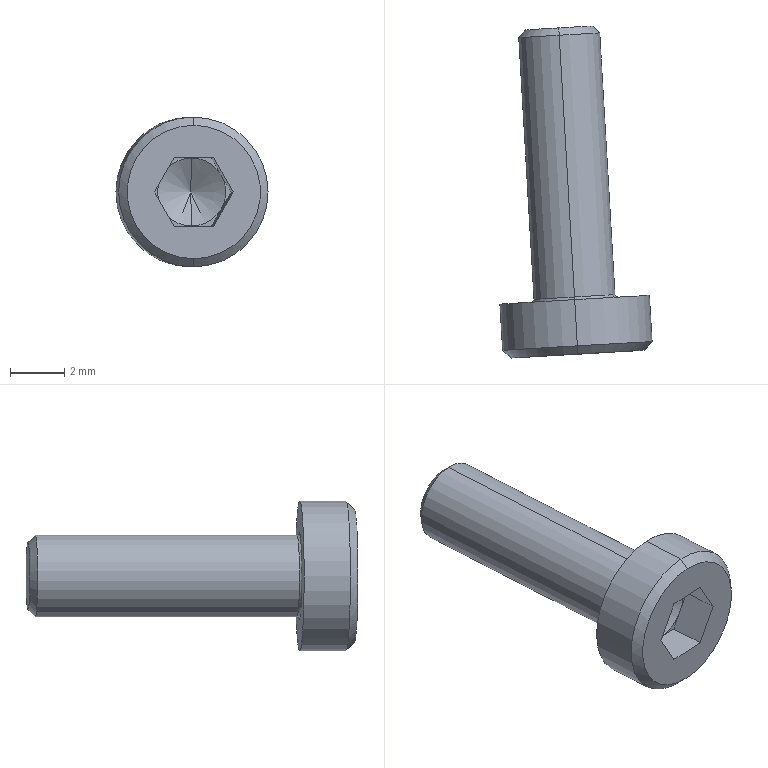Component | SolidWorks | MotorAssemblyWhen2-1_MCOCG20-8-10-1_M3-10_bo2-1 | 1 solid | 27 faces | box 5.59 x 12.19 x 5.5 mm | volume 109 mm3 | plane 15 | cone 6 | cylinder 4 | spline 2 | commonest cylinder face diameters 3 x2 5.5 x2
STEP:
#1=COLOUR_RGB('',0.7922,0.8196,0.9333);
#2=FILL_AREA_STYLE_COLOUR('',#1);
#3=FILL_AREA_STYLE('',(#2));
#4=SURFACE_STYLE_FILL_AREA(#3);
#5=SURFACE_SIDE_STYLE('',(#4));
#6=SURFACE_STYLE_USAGE(.BOTH.,#5);
#7=PRESENTATION_STYLE_ASSIGNMENT((#6));
#8=CARTESIAN_POINT('',(-2.236,5.18,-4.868));
#9=VERTEX_POINT('',#8);
#10=CARTESIAN_POINT('',(-2.236,5.18,-4.986));
#11=VERTEX_POINT('',#10);
#12=CARTESIAN_POINT('',(-2.236,5.18,-4.927));
#13=DIRECTION('',(-0.05821,0.9983,0.));
#14=DIRECTION('',(0.,0.,-1.));
#15=AXIS2_PLACEMENT_3D('',#12,#13,#14);
#16=CIRCLE('',#15,0.05906);
#17=EDGE_CURVE('',#9,#11,#16,.T.);
#18=ORIENTED_EDGE('',*,*,#17,.F.);
#19=CARTESIAN_POINT('',(-2.235,5.176,-4.864));
#20=VERTEX_POINT('',#19);
#21=CARTESIAN_POINT('',(-2.236,5.18,-4.864));
#22=DIRECTION('',(-0.9983,-0.05821,0.));
#23=DIRECTION('',(0.,0.,1.));
#24=AXIS2_PLACEMENT_3D('',#21,#22,#23);
#25=CIRCLE('',#24,0.003937);
#26=EDGE_CURVE('',#9,#20,#25,.T.);
#27=ORIENTED_EDGE('',*,*,#26,.T.);
#28=CARTESIAN_POINT('',(-2.235,5.176,-4.99));
#29=VERTEX_POINT('',#28);
#30=CARTESIAN_POINT('',(-2.235,5.176,-4.99));
#31=CARTESIAN_POINT('',(-2.231,5.176,-4.99));
#32=CARTESIAN_POINT('',(-2.225,5.177,-4.99));
#33=CARTESIAN_POINT('',(-2.219,5.177,-4.988));
#34=CARTESIAN_POINT('',(-2.215,5.177,-4.987));
#35=CARTESIAN_POINT('',(-2.214,5.177,-4.987));
#36=CARTESIAN_POINT('',(-2.213,5.177,-4.986));
#37=CARTESIAN_POINT('',(-2.213,5.177,-4.986));
#38=CARTESIAN_POINT('',(-2.204,5.178,-4.983));
#39=CARTESIAN_POINT('',(-2.197,5.178,-4.978));
#40=CARTESIAN_POINT('',(-2.188,5.179,-4.969));
#41=CARTESIAN_POINT('',(-2.184,5.179,-4.964));
#42=CARTESIAN_POINT('',(-2.18,5.179,-4.957));
#43=CARTESIAN_POINT('',(-2.179,5.179,-4.955));
#44=CARTESIAN_POINT('',(-2.178,5.179,-4.953));
#45=CARTESIAN_POINT('',(-2.177,5.179,-4.951));
#46=CARTESIAN_POINT('',(-2.174,5.18,-4.943));
#47=CARTESIAN_POINT('',(-2.172,5.18,-4.935));
#48=CARTESIAN_POINT('',(-2.172,5.18,-4.923));
#49=CARTESIAN_POINT('',(-2.173,5.18,-4.917));
#50=CARTESIAN_POINT('',(-2.175,5.179,-4.911));
#51=CARTESIAN_POINT('',(-2.176,5.179,-4.907));
#52=CARTESIAN_POINT('',(-2.176,5.179,-4.906));
#53=CARTESIAN_POINT('',(-2.176,5.179,-4.905));
#54=CARTESIAN_POINT('',(-2.177,5.179,-4.905));
#55=CARTESIAN_POINT('',(-2.18,5.179,-4.896));
#56=CARTESIAN_POINT('',(-2.185,5.179,-4.889));
#57=CARTESIAN_POINT('',(-2.194,5.178,-4.88));
#58=CARTESIAN_POINT('',(-2.199,5.178,-4.876));
#59=CARTESIAN_POINT('',(-2.205,5.178,-4.872));
#60=CARTESIAN_POINT('',(-2.208,5.178,-4.871));
#61=CARTESIAN_POINT('',(-2.21,5.177,-4.87));
#62=CARTESIAN_POINT('',(-2.211,5.177,-4.869));
#63=CARTESIAN_POINT('',(-2.22,5.177,-4.866));
#64=CARTESIAN_POINT('',(-2.227,5.176,-4.864));
#65=CARTESIAN_POINT('',(-2.235,5.176,-4.864));
#66=B_SPLINE_CURVE_WITH_KNOTS('',3,(#30,#31,#32,#33,#34,#35,#36,#37,#38,#39,#40,#41,#42,#43,#44,#45,#46,#47,#48,#49,#50,#51,#52,#53,#54,#55,#56,#57,#58,#59,#60,#61,#62,#63,#64,#65),.UNSPECIFIED.,.F.,.F.,(4,1,1,1,2,2,2,1,1,2,2,2,1,1,1,2,2,2,1,1,2,2,4),(0.,0.0625,0.09375,0.1094,0.1172,0.125,0.25,0.3125,0.3438,0.3594,0.375,0.5,0.5625,0.5938,0.6094,0.6172,0.625,0.75,0.8125,0.8438,0.8594,0.875,1.),.UNSPECIFIED.);
#67=EDGE_CURVE('',#29,#20,#66,.T.);
#68=ORIENTED_EDGE('',*,*,#67,.F.);
#69=CARTESIAN_POINT('',(-2.236,5.18,-4.99));
#70=DIRECTION('',(0.9983,0.05821,0.));
#71=DIRECTION('',(0.,0.,-1.));
#72=AXIS2_PLACEMENT_3D('',#69,#70,#71);
#73=CIRCLE('',#72,0.003937);
#74=EDGE_CURVE('',#11,#29,#73,.T.);
#75=ORIENTED_EDGE('',*,*,#74,.F.);
#76=EDGE_LOOP('',(#18,#27,#68,#75));
#77=FACE_OUTER_BOUND('',#76,.T.);
#78=CARTESIAN_POINT('',(-2.236,5.18,-4.986));
#79=CARTESIAN_POINT('',(-2.118,5.187,-4.986));
#80=CARTESIAN_POINT('',(-2.118,5.187,-4.868));
#81=CARTESIAN_POINT('',(-2.236,5.18,-4.868));
#82=CARTESIAN_POINT('',(-2.235,5.178,-4.986));
#83=CARTESIAN_POINT('',(-2.117,5.184,-4.986));
#84=CARTESIAN_POINT('',(-2.117,5.184,-4.868));
#85=CARTESIAN_POINT('',(-2.235,5.178,-4.868));
#86=CARTESIAN_POINT('',(-2.235,5.176,-4.988));
#87=CARTESIAN_POINT('',(-2.114,5.183,-4.988));
#88=CARTESIAN_POINT('',(-2.114,5.183,-4.867));
#89=CARTESIAN_POINT('',(-2.235,5.176,-4.867));
#90=CARTESIAN_POINT('',(-2.235,5.176,-4.99));
#91=CARTESIAN_POINT('',(-2.11,5.183,-4.99));
#92=CARTESIAN_POINT('',(-2.11,5.183,-4.864));
#93=CARTESIAN_POINT('',(-2.235,5.176,-4.864));
#94=(BOUNDED_SURFACE()B_SPLINE_SURFACE(3,3,((#78,#79,#80,#81),(#82,#83,#84,#85),(#86,#87,#88,#89),(#90,#91,#92,#93)),.UNSPECIFIED.,.F.,.F.,.T.)B_SPLINE_SURFACE_WITH_KNOTS((4,4),(4,4),(0.,1.),(0.,1.),.UNSPECIFIED.)GEOMETRIC_REPRESENTATION_ITEM()RATIONAL_B_SPLINE_SURFACE(((1.,0.3333,0.3333,1.),(0.8047,0.2682,0.2682,0.8047),(0.8047,0.2682,0.2682,0.8047),(1.,0.3333,0.3333,1.)))REPRESENTATION_ITEM('')SURFACE());
#95=ADVANCED_FACE('',(#77),#94,.F.);
#96=CARTESIAN_POINT('',(-2.258,5.558,-4.986));
#97=VERTEX_POINT('',#96);
#98=CARTESIAN_POINT('',(-2.258,5.558,-4.868));
#99=VERTEX_POINT('',#98);
#100=CARTESIAN_POINT('',(-2.258,5.558,-4.927));
#101=DIRECTION('',(0.05821,-0.9983,-0.));
#102=DIRECTION('',(0.,0.,-1.));
#103=AXIS2_PLACEMENT_3D('',#100,#101,#102);
#104=CIRCLE('',#103,0.05906);
#105=EDGE_CURVE('',#97,#99,#104,.T.);
#106=ORIENTED_EDGE('',*,*,#105,.T.);
#107=CARTESIAN_POINT('',(-2.258,5.569,-4.868));
#108=DIRECTION('',(0.05821,-0.9983,-0.));
#109=VECTOR('',#108,39.37);
#110=LINE('',#107,#109);
#111=EDGE_CURVE('',#99,#9,#110,.T.);
#112=ORIENTED_EDGE('',*,*,#111,.T.);
#113=ORIENTED_EDGE('',*,*,#17,.T.);
#114=CARTESIAN_POINT('',(-2.258,5.569,-4.986));
#115=DIRECTION('',(0.05821,-0.9983,-0.));
#116=VECTOR('',#115,39.37);
#117=LINE('',#114,#116);
#118=EDGE_CURVE('',#97,#11,#117,.T.);
#119=ORIENTED_EDGE('',*,*,#118,.F.);
#120=EDGE_LOOP('',(#106,#112,#113,#119));
#121=FACE_OUTER_BOUND('',#120,.T.);
#122=CARTESIAN_POINT('',(-2.258,5.569,-4.927));
#123=DIRECTION('',(0.05821,-0.9983,-0.));
#124=DIRECTION('',(0.,0.,-1.));
#125=AXIS2_PLACEMENT_3D('',#122,#123,#124);
#126=CYLINDRICAL_SURFACE('',#125,0.05906);
#127=ADVANCED_FACE('',(#121),#126,.T.);
#128=CARTESIAN_POINT('',(-2.258,5.569,-4.976));
#129=VERTEX_POINT('',#128);
#130=CARTESIAN_POINT('',(-2.258,5.569,-4.879));
#131=VERTEX_POINT('',#130);
#132=CARTESIAN_POINT('',(-2.258,5.569,-4.927));
#133=DIRECTION('',(0.05821,-0.9983,-0.));
#134=DIRECTION('',(0.,0.,-1.));
#135=AXIS2_PLACEMENT_3D('',#132,#133,#134);
#136=CIRCLE('',#135,0.04841);
#137=EDGE_CURVE('',#129,#131,#136,.T.);
#138=ORIENTED_EDGE('',*,*,#137,.T.);
#139=CARTESIAN_POINT('',(-2.258,5.558,-4.868));
#140=DIRECTION('',(0.04116,-0.7059,0.7071));
#141=VECTOR('',#140,39.37);
#142=LINE('',#139,#141);
#143=EDGE_CURVE('',#131,#99,#142,.T.);
#144=ORIENTED_EDGE('',*,*,#143,.T.);
#145=ORIENTED_EDGE('',*,*,#105,.F.);
#146=CARTESIAN_POINT('',(-2.258,5.558,-4.986));
#147=DIRECTION('',(0.04116,-0.7059,-0.7071));
#148=VECTOR('',#147,39.37);
#149=LINE('',#146,#148);
#150=EDGE_CURVE('',#129,#97,#149,.T.);
#151=ORIENTED_EDGE('',*,*,#150,.F.);
#152=EDGE_LOOP('',(#138,#144,#145,#151));
#153=FACE_OUTER_BOUND('',#152,.T.);
#154=CARTESIAN_POINT('',(-2.258,5.558,-4.927));
#155=DIRECTION('',(0.05821,-0.9983,-0.));
#156=DIRECTION('',(0.,0.,-1.));
#157=AXIS2_PLACEMENT_3D('',#154,#155,#156);
#158=CONICAL_SURFACE('',#157,0.05906,0.7854);
#159=ADVANCED_FACE('',(#153),#158,.T.);
#160=CARTESIAN_POINT('',(-2.235,5.176,-5.036));
#161=VERTEX_POINT('',#160);
#162=CARTESIAN_POINT('',(-2.235,5.176,-4.819));
#163=VERTEX_POINT('',#162);
#164=CARTESIAN_POINT('',(-2.235,5.176,-4.927));
#165=DIRECTION('',(0.05821,-0.9983,-0.));
#166=DIRECTION('',(0.,0.,-1.));
#167=AXIS2_PLACEMENT_3D('',#164,#165,#166);
#168=CIRCLE('',#167,0.1083);
#169=EDGE_CURVE('',#161,#163,#168,.T.);
#170=ORIENTED_EDGE('',*,*,#169,.T.);
#171=CARTESIAN_POINT('',(-2.231,5.109,-4.819));
#172=VERTEX_POINT('',#171);
#173=CARTESIAN_POINT('',(-2.258,5.569,-4.819));
#174=DIRECTION('',(0.05821,-0.9983,-0.));
#175=VECTOR('',#174,39.37);
#176=LINE('',#173,#175);
#177=EDGE_CURVE('',#163,#172,#176,.T.);
#178=ORIENTED_EDGE('',*,*,#177,.T.);
#179=CARTESIAN_POINT('',(-2.231,5.109,-5.036));
#180=VERTEX_POINT('',#179);
#181=CARTESIAN_POINT('',(-2.231,5.109,-4.927));
#182=DIRECTION('',(-0.05821,0.9983,0.));
#183=DIRECTION('',(-0.,0.,-1.));
#184=AXIS2_PLACEMENT_3D('',#181,#182,#183);
#185=CIRCLE('',#184,0.1083);
#186=EDGE_CURVE('',#172,#180,#185,.T.);
#187=ORIENTED_EDGE('',*,*,#186,.T.);
#188=CARTESIAN_POINT('',(-2.258,5.569,-5.036));
#189=DIRECTION('',(0.05821,-0.9983,-0.));
#190=VECTOR('',#189,39.37);
#191=LINE('',#188,#190);
#192=EDGE_CURVE('',#161,#180,#191,.T.);
#193=ORIENTED_EDGE('',*,*,#192,.F.);
#194=EDGE_LOOP('',(#170,#178,#187,#193));
#195=FACE_OUTER_BOUND('',#194,.T.);
#196=CARTESIAN_POINT('',(-2.258,5.569,-4.927));
#197=DIRECTION('',(0.05821,-0.9983,-0.));
#198=DIRECTION('',(0.,0.,-1.));
#199=AXIS2_PLACEMENT_3D('',#196,#197,#198);
#200=CYLINDRICAL_SURFACE('',#199,0.1083);
#201=ADVANCED_FACE('',(#195),#200,.T.);
#202=CARTESIAN_POINT('',(-2.231,5.097,-4.831));
#203=VERTEX_POINT('',#202);
#204=CARTESIAN_POINT('',(-2.231,5.097,-5.024));
#205=VERTEX_POINT('',#204);
#206=CARTESIAN_POINT('',(-2.231,5.097,-4.927));
#207=DIRECTION('',(-0.05821,0.9983,0.));
#208=DIRECTION('',(0.,0.,1.));
#209=AXIS2_PLACEMENT_3D('',#206,#207,#208);
#210=CIRCLE('',#209,0.09646);
#211=EDGE_CURVE('',#203,#205,#210,.T.);
#212=ORIENTED_EDGE('',*,*,#211,.T.);
#213=CARTESIAN_POINT('',(-2.231,5.109,-5.036));
#214=DIRECTION('',(-0.04116,0.7059,-0.7071));
#215=VECTOR('',#214,39.37);
#216=LINE('',#213,#215);
#217=EDGE_CURVE('',#205,#180,#216,.T.);
#218=ORIENTED_EDGE('',*,*,#217,.T.);
#219=ORIENTED_EDGE('',*,*,#186,.F.);
#220=CARTESIAN_POINT('',(-2.231,5.109,-4.819));
#221=DIRECTION('',(-0.04116,0.7059,0.7071));
#222=VECTOR('',#221,39.37);
#223=LINE('',#220,#222);
#224=EDGE_CURVE('',#203,#172,#223,.T.);
#225=ORIENTED_EDGE('',*,*,#224,.F.);
#226=EDGE_LOOP('',(#212,#218,#219,#225));
#227=FACE_OUTER_BOUND('',#226,.T.);
#228=CARTESIAN_POINT('',(-2.231,5.109,-4.927));
#229=DIRECTION('',(-0.05821,0.9983,0.));
#230=DIRECTION('',(0.,0.,1.));
#231=AXIS2_PLACEMENT_3D('',#228,#229,#230);
#232=CONICAL_SURFACE('',#231,0.1083,0.7854);
#233=ADVANCED_FACE('',(#227),#232,.T.);
#234=CARTESIAN_POINT('',(-2.235,5.177,-4.927));
#235=VERTEX_POINT('',#234);
#236=CARTESIAN_POINT('',(-2.234,5.148,-4.977));
#237=VERTEX_POINT('',#236);
#238=CARTESIAN_POINT('',(-2.234,5.148,-4.977));
#239=DIRECTION('',(0.0291,-0.4992,-0.866));
#240=VECTOR('',#239,39.37);
#241=LINE('',#238,#240);
#242=EDGE_CURVE('',#235,#237,#241,.T.);
#243=ORIENTED_EDGE('',*,*,#242,.F.);
#244=CARTESIAN_POINT('',(-2.234,5.148,-4.878));
#245=VERTEX_POINT('',#244);
#246=CARTESIAN_POINT('',(-2.234,5.148,-4.878));
#247=DIRECTION('',(0.0291,-0.4992,0.866));
#248=VECTOR('',#247,39.37);
#249=LINE('',#246,#248);
#250=EDGE_CURVE('',#235,#245,#249,.T.);
#251=ORIENTED_EDGE('',*,*,#250,.T.);
#252=CARTESIAN_POINT('',(-2.276,5.146,-4.903));
#253=VERTEX_POINT('',#252);
#254=CARTESIAN_POINT('',(-2.234,5.148,-4.927));
#255=DIRECTION('',(0.05821,-0.9983,-0.));
#256=DIRECTION('',(0.,0.,-1.));
#257=AXIS2_PLACEMENT_3D('',#254,#255,#256);
#258=CIRCLE('',#257,0.04921);
#259=EDGE_CURVE('',#245,#253,#258,.T.);
#260=ORIENTED_EDGE('',*,*,#259,.T.);
#261=CARTESIAN_POINT('',(-2.276,5.146,-4.952));
#262=VERTEX_POINT('',#261);
#263=CARTESIAN_POINT('',(-2.234,5.148,-4.927));
#264=DIRECTION('',(0.05821,-0.9983,-0.));
#265=DIRECTION('',(0.,0.,-1.));
#266=AXIS2_PLACEMENT_3D('',#263,#264,#265);
#267=CIRCLE('',#266,0.04921);
#268=EDGE_CURVE('',#253,#262,#267,.T.);
#269=ORIENTED_EDGE('',*,*,#268,.T.);
#270=CARTESIAN_POINT('',(-2.234,5.148,-4.927));
#271=DIRECTION('',(0.05821,-0.9983,-0.));
#272=DIRECTION('',(0.,0.,-1.));
#273=AXIS2_PLACEMENT_3D('',#270,#271,#272);
#274=CIRCLE('',#273,0.04921);
#275=EDGE_CURVE('',#262,#237,#274,.T.);
#276=ORIENTED_EDGE('',*,*,#275,.T.);
#277=EDGE_LOOP('',(#243,#251,#260,#269,#276));
#278=FACE_OUTER_BOUND('',#277,.T.);
#279=CARTESIAN_POINT('',(-2.234,5.148,-4.927));
#280=DIRECTION('',(0.05821,-0.9983,-0.));
#281=DIRECTION('',(0.,0.,-1.));
#282=AXIS2_PLACEMENT_3D('',#279,#280,#281);
#283=CONICAL_SURFACE('',#282,0.04921,1.047);
#284=ADVANCED_FACE('',(#278),#283,.F.);
#285=ORIENTED_EDGE('',*,*,#111,.F.);
#286=CARTESIAN_POINT('',(-2.258,5.558,-4.927));
#287=DIRECTION('',(0.05821,-0.9983,-0.));
#288=DIRECTION('',(0.,0.,-1.));
#289=AXIS2_PLACEMENT_3D('',#286,#287,#288);
#290=CIRCLE('',#289,0.05906);
#291=EDGE_CURVE('',#99,#97,#290,.T.);
#292=ORIENTED_EDGE('',*,*,#291,.T.);
#293=ORIENTED_EDGE('',*,*,#118,.T.);
#294=CARTESIAN_POINT('',(-2.236,5.18,-4.927));
#295=DIRECTION('',(-0.05821,0.9983,0.));
#296=DIRECTION('',(0.,0.,-1.));
#297=AXIS2_PLACEMENT_3D('',#294,#295,#296);
#298=CIRCLE('',#297,0.05906);
#299=EDGE_CURVE('',#11,#9,#298,.T.);
#300=ORIENTED_EDGE('',*,*,#299,.T.);
#301=EDGE_LOOP('',(#285,#292,#293,#300));
#302=FACE_OUTER_BOUND('',#301,.T.);
#303=CARTESIAN_POINT('',(-2.258,5.569,-4.927));
#304=DIRECTION('',(0.05821,-0.9983,-0.));
#305=DIRECTION('',(0.,0.,-1.));
#306=AXIS2_PLACEMENT_3D('',#303,#304,#305);
#307=CYLINDRICAL_SURFACE('',#306,0.05906);
#308=ADVANCED_FACE('',(#302),#307,.T.);
#309=ORIENTED_EDGE('',*,*,#26,.F.);
#310=ORIENTED_EDGE('',*,*,#299,.F.);
#311=ORIENTED_EDGE('',*,*,#74,.T.);
#312=CARTESIAN_POINT('',(-2.235,5.176,-4.864));
#313=CARTESIAN_POINT('',(-2.239,5.176,-4.864));
#314=CARTESIAN_POINT('',(-2.245,5.175,-4.865));
#315=CARTESIAN_POINT('',(-2.252,5.175,-4.867));
#316=CARTESIAN_POINT('',(-2.255,5.175,-4.868));
#317=CARTESIAN_POINT('',(-2.257,5.175,-4.868));
#318=CARTESIAN_POINT('',(-2.258,5.175,-4.868));
#319=CARTESIAN_POINT('',(-2.258,5.175,-4.869));
#320=CARTESIAN_POINT('',(-2.267,5.174,-4.872));
#321=CARTESIAN_POINT('',(-2.274,5.174,-4.877));
#322=CARTESIAN_POINT('',(-2.283,5.173,-4.886));
#323=CARTESIAN_POINT('',(-2.287,5.173,-4.891));
#324=CARTESIAN_POINT('',(-2.291,5.173,-4.897));
#325=CARTESIAN_POINT('',(-2.292,5.173,-4.9));
#326=CARTESIAN_POINT('',(-2.293,5.173,-4.902));
#327=CARTESIAN_POINT('',(-2.293,5.173,-4.903));
#328=CARTESIAN_POINT('',(-2.297,5.172,-4.912));
#329=CARTESIAN_POINT('',(-2.298,5.172,-4.919));
#330=CARTESIAN_POINT('',(-2.298,5.172,-4.931));
#331=CARTESIAN_POINT('',(-2.298,5.172,-4.937));
#332=CARTESIAN_POINT('',(-2.296,5.172,-4.944));
#333=CARTESIAN_POINT('',(-2.295,5.172,-4.947));
#334=CARTESIAN_POINT('',(-2.294,5.172,-4.949));
#335=CARTESIAN_POINT('',(-2.294,5.173,-4.95));
#336=CARTESIAN_POINT('',(-2.294,5.173,-4.95));
#337=CARTESIAN_POINT('',(-2.291,5.173,-4.959));
#338=CARTESIAN_POINT('',(-2.286,5.173,-4.966));
#339=CARTESIAN_POINT('',(-2.277,5.174,-4.975));
#340=CARTESIAN_POINT('',(-2.272,5.174,-4.979));
#341=CARTESIAN_POINT('',(-2.265,5.174,-4.983));
#342=CARTESIAN_POINT('',(-2.262,5.174,-4.984));
#343=CARTESIAN_POINT('',(-2.26,5.174,-4.985));
#344=CARTESIAN_POINT('',(-2.259,5.175,-4.986));
#345=CARTESIAN_POINT('',(-2.251,5.175,-4.989));
#346=CARTESIAN_POINT('',(-2.243,5.175,-4.99));
#347=CARTESIAN_POINT('',(-2.235,5.176,-4.99));
#348=B_SPLINE_CURVE_WITH_KNOTS('',3,(#312,#313,#314,#315,#316,#317,#318,#319,#320,#321,#322,#323,#324,#325,#326,#327,#328,#329,#330,#331,#332,#333,#334,#335,#336,#337,#338,#339,#340,#341,#342,#343,#344,#345,#346,#347),.UNSPECIFIED.,.F.,.F.,(4,1,1,1,2,2,2,1,1,2,2,2,1,1,1,2,2,2,1,1,2,2,4),(0.,0.0625,0.09375,0.1094,0.1172,0.125,0.25,0.3125,0.3438,0.3594,0.375,0.5,0.5625,0.5938,0.6094,0.6172,0.625,0.75,0.8125,0.8438,0.8594,0.875,1.),.UNSPECIFIED.);
#349=EDGE_CURVE('',#20,#29,#348,.T.);
#350=ORIENTED_EDGE('',*,*,#349,.F.);
#351=EDGE_LOOP('',(#309,#310,#311,#350));
#352=FACE_OUTER_BOUND('',#351,.T.);
#353=CARTESIAN_POINT('',(-2.236,5.18,-4.868));
#354=CARTESIAN_POINT('',(-2.353,5.173,-4.868));
#355=CARTESIAN_POINT('',(-2.353,5.173,-4.986));
#356=CARTESIAN_POINT('',(-2.236,5.18,-4.986));
#357=CARTESIAN_POINT('',(-2.235,5.178,-4.868));
#358=CARTESIAN_POINT('',(-2.353,5.171,-4.868));
#359=CARTESIAN_POINT('',(-2.353,5.171,-4.986));
#360=CARTESIAN_POINT('',(-2.235,5.178,-4.986));
#361=CARTESIAN_POINT('',(-2.235,5.176,-4.867));
#362=CARTESIAN_POINT('',(-2.356,5.169,-4.867));
#363=CARTESIAN_POINT('',(-2.356,5.169,-4.988));
#364=CARTESIAN_POINT('',(-2.235,5.176,-4.988));
#365=CARTESIAN_POINT('',(-2.235,5.176,-4.864));
#366=CARTESIAN_POINT('',(-2.361,5.169,-4.864));
#367=CARTESIAN_POINT('',(-2.361,5.169,-4.99));
#368=CARTESIAN_POINT('',(-2.235,5.176,-4.99));
#369=(BOUNDED_SURFACE()B_SPLINE_SURFACE(3,3,((#353,#354,#355,#356),(#357,#358,#359,#360),(#361,#362,#363,#364),(#365,#366,#367,#368)),.UNSPECIFIED.,.F.,.F.,.T.)B_SPLINE_SURFACE_WITH_KNOTS((4,4),(4,4),(0.,1.),(0.,1.),.UNSPECIFIED.)GEOMETRIC_REPRESENTATION_ITEM()RATIONAL_B_SPLINE_SURFACE(((1.,0.3333,0.3333,1.),(0.8047,0.2682,0.2682,0.8047),(0.8047,0.2682,0.2682,0.8047),(1.,0.3333,0.3333,1.)))REPRESENTATION_ITEM('')SURFACE());
#370=ADVANCED_FACE('',(#352),#369,.F.);
#371=ORIENTED_EDGE('',*,*,#143,.F.);
#372=CARTESIAN_POINT('',(-2.258,5.569,-4.927));
#373=DIRECTION('',(0.05821,-0.9983,-0.));
#374=DIRECTION('',(0.,0.,-1.));
#375=AXIS2_PLACEMENT_3D('',#372,#373,#374);
#376=CIRCLE('',#375,0.04841);
#377=EDGE_CURVE('',#131,#129,#376,.T.);
#378=ORIENTED_EDGE('',*,*,#377,.T.);
#379=ORIENTED_EDGE('',*,*,#150,.T.);
#380=ORIENTED_EDGE('',*,*,#291,.F.);
#381=EDGE_LOOP('',(#371,#378,#379,#380));
#382=FACE_OUTER_BOUND('',#381,.T.);
#383=CARTESIAN_POINT('',(-2.258,5.558,-4.927));
#384=DIRECTION('',(0.05821,-0.9983,-0.));
#385=DIRECTION('',(0.,0.,-1.));
#386=AXIS2_PLACEMENT_3D('',#383,#384,#385);
#387=CONICAL_SURFACE('',#386,0.05906,0.7854);
#388=ADVANCED_FACE('',(#382),#387,.T.);
#389=ORIENTED_EDGE('',*,*,#349,.T.);
#390=ORIENTED_EDGE('',*,*,#67,.T.);
#391=EDGE_LOOP('',(#389,#390));
#392=FACE_BOUND('',#391,.T.);
#393=ORIENTED_EDGE('',*,*,#169,.F.);
#394=CARTESIAN_POINT('',(-2.235,5.176,-4.927));
#395=DIRECTION('',(0.05821,-0.9983,-0.));
#396=DIRECTION('',(0.,0.,-1.));
#397=AXIS2_PLACEMENT_3D('',#394,#395,#396);
#398=CIRCLE('',#397,0.1083);
#399=EDGE_CURVE('',#163,#161,#398,.T.);
#400=ORIENTED_EDGE('',*,*,#399,.F.);
#401=EDGE_LOOP('',(#393,#400));
#402=FACE_OUTER_BOUND('',#401,.T.);
#403=CARTESIAN_POINT('',(-2.127,5.182,-4.927));
#404=DIRECTION('',(0.05821,-0.9983,-0.));
#405=DIRECTION('',(-0.,0.,-1.));
#406=AXIS2_PLACEMENT_3D('',#403,#404,#405);
#407=PLANE('',#406);
#408=ADVANCED_FACE('',(#392,#402),#407,.F.);
#409=ORIENTED_EDGE('',*,*,#137,.F.);
#410=ORIENTED_EDGE('',*,*,#377,.F.);
#411=EDGE_LOOP('',(#409,#410));
#412=FACE_OUTER_BOUND('',#411,.T.);
#413=CARTESIAN_POINT('',(-2.21,5.572,-4.927));
#414=DIRECTION('',(0.05821,-0.9983,-0.));
#415=DIRECTION('',(-0.,0.,-1.));
#416=AXIS2_PLACEMENT_3D('',#413,#414,#415);
#417=PLANE('',#416);
#418=ADVANCED_FACE('',(#412),#417,.F.);
#419=ORIENTED_EDGE('',*,*,#177,.F.);
#420=ORIENTED_EDGE('',*,*,#399,.T.);
#421=ORIENTED_EDGE('',*,*,#192,.T.);
#422=CARTESIAN_POINT('',(-2.231,5.109,-4.927));
#423=DIRECTION('',(-0.05821,0.9983,0.));
#424=DIRECTION('',(0.,0.,-1.));
#425=AXIS2_PLACEMENT_3D('',#422,#423,#424);
#426=CIRCLE('',#425,0.1083);
#427=EDGE_CURVE('',#180,#172,#426,.T.);
#428=ORIENTED_EDGE('',*,*,#427,.T.);
#429=EDGE_LOOP('',(#419,#420,#421,#428));
#430=FACE_OUTER_BOUND('',#429,.T.);
#431=CARTESIAN_POINT('',(-2.258,5.569,-4.927));
#432=DIRECTION('',(0.05821,-0.9983,-0.));
#433=DIRECTION('',(0.,0.,-1.));
#434=AXIS2_PLACEMENT_3D('',#431,#432,#433);
#435=CYLINDRICAL_SURFACE('',#434,0.1083);
#436=ADVANCED_FACE('',(#430),#435,.T.);
#437=ORIENTED_EDGE('',*,*,#217,.F.);
#438=CARTESIAN_POINT('',(-2.231,5.097,-4.927));
#439=DIRECTION('',(-0.05821,0.9983,0.));
#440=DIRECTION('',(0.,0.,1.));
#441=AXIS2_PLACEMENT_3D('',#438,#439,#440);
#442=CIRCLE('',#441,0.09646);
#443=EDGE_CURVE('',#205,#203,#442,.T.);
#444=ORIENTED_EDGE('',*,*,#443,.T.);
#445=ORIENTED_EDGE('',*,*,#224,.T.);
#446=ORIENTED_EDGE('',*,*,#427,.F.);
#447=EDGE_LOOP('',(#437,#444,#445,#446));
#448=FACE_OUTER_BOUND('',#447,.T.);
#449=CARTESIAN_POINT('',(-2.231,5.109,-4.927));
#450=DIRECTION('',(-0.05821,0.9983,0.));
#451=DIRECTION('',(0.,0.,1.));
#452=AXIS2_PLACEMENT_3D('',#449,#450,#451);
#453=CONICAL_SURFACE('',#452,0.1083,0.7854);
#454=ADVANCED_FACE('',(#448),#453,.T.);
#455=CARTESIAN_POINT('',(-2.259,5.096,-4.977));
#456=VERTEX_POINT('',#455);
#457=CARTESIAN_POINT('',(-2.202,5.099,-4.977));
#458=VERTEX_POINT('',#457);
#459=CARTESIAN_POINT('',(-2.231,5.097,-4.977));
#460=DIRECTION('',(0.9983,0.05821,0.));
#461=VECTOR('',#460,39.37);
#462=LINE('',#459,#461);
#463=EDGE_CURVE('',#456,#458,#462,.T.);
#464=ORIENTED_EDGE('',*,*,#463,.F.);
#465=CARTESIAN_POINT('',(-2.287,5.094,-4.927));
#466=VERTEX_POINT('',#465);
#467=CARTESIAN_POINT('',(-2.287,5.094,-4.927));
#468=DIRECTION('',(0.4992,0.0291,-0.866));
#469=VECTOR('',#468,39.37);
#470=LINE('',#467,#469);
#471=EDGE_CURVE('',#466,#456,#470,.T.);
#472=ORIENTED_EDGE('',*,*,#471,.F.);
#473=CARTESIAN_POINT('',(-2.259,5.096,-4.878));
#474=VERTEX_POINT('',#473);
#475=CARTESIAN_POINT('',(-2.259,5.096,-4.878));
#476=DIRECTION('',(-0.4992,-0.0291,-0.866));
#477=VECTOR('',#476,39.37);
#478=LINE('',#475,#477);
#479=EDGE_CURVE('',#474,#466,#478,.T.);
#480=ORIENTED_EDGE('',*,*,#479,.F.);
#481=CARTESIAN_POINT('',(-2.202,5.099,-4.878));
#482=VERTEX_POINT('',#481);
#483=CARTESIAN_POINT('',(-2.231,5.097,-4.878));
#484=DIRECTION('',(-0.9983,-0.05821,-0.));
#485=VECTOR('',#484,39.37);
#486=LINE('',#483,#485);
#487=EDGE_CURVE('',#482,#474,#486,.T.);
#488=ORIENTED_EDGE('',*,*,#487,.F.);
#489=CARTESIAN_POINT('',(-2.174,5.101,-4.927));
#490=VERTEX_POINT('',#489);
#491=CARTESIAN_POINT('',(-2.174,5.101,-4.927));
#492=DIRECTION('',(-0.4992,-0.0291,0.866));
#493=VECTOR('',#492,39.37);
#494=LINE('',#491,#493);
#495=EDGE_CURVE('',#490,#482,#494,.T.);
#496=ORIENTED_EDGE('',*,*,#495,.F.);
#497=CARTESIAN_POINT('',(-2.202,5.099,-4.977));
#498=DIRECTION('',(0.4992,0.0291,0.866));
#499=VECTOR('',#498,39.37);
#500=LINE('',#497,#499);
#501=EDGE_CURVE('',#458,#490,#500,.T.);
#502=ORIENTED_EDGE('',*,*,#501,.F.);
#503=EDGE_LOOP('',(#464,#472,#480,#488,#496,#502));
#504=FACE_BOUND('',#503,.T.);
#505=ORIENTED_EDGE('',*,*,#211,.F.);
#506=ORIENTED_EDGE('',*,*,#443,.F.);
#507=EDGE_LOOP('',(#505,#506));
#508=FACE_OUTER_BOUND('',#507,.T.);
#509=CARTESIAN_POINT('',(-2.231,5.097,-4.927));
#510=DIRECTION('',(-0.05821,0.9983,0.));
#511=DIRECTION('',(0.,-0.,1.));
#512=AXIS2_PLACEMENT_3D('',#509,#510,#511);
#513=PLANE('',#512);
#514=ADVANCED_FACE('',(#504,#508),#513,.F.);
#515=CARTESIAN_POINT('',(-2.191,5.151,-4.952));
#516=VERTEX_POINT('',#515);
#517=CARTESIAN_POINT('',(-2.205,5.15,-4.977));
#518=VERTEX_POINT('',#517);
#519=CARTESIAN_POINT('',(-2.177,5.152,-4.927));
#520=DIRECTION('',(-0.4992,-0.0291,-0.866));
#521=VECTOR('',#520,39.37);
#522=LINE('',#519,#521);
#523=EDGE_CURVE('',#516,#518,#522,.T.);
#524=ORIENTED_EDGE('',*,*,#523,.T.);
#525=CARTESIAN_POINT('',(-2.205,5.15,-4.977));
#526=DIRECTION('',(0.05821,-0.9983,-0.));
#527=VECTOR('',#526,39.37);
#528=LINE('',#525,#527);
#529=EDGE_CURVE('',#518,#458,#528,.T.);
#530=ORIENTED_EDGE('',*,*,#529,.T.);
#531=ORIENTED_EDGE('',*,*,#501,.T.);
#532=CARTESIAN_POINT('',(-2.177,5.152,-4.927));
#533=VERTEX_POINT('',#532);
#534=CARTESIAN_POINT('',(-2.177,5.152,-4.927));
#535=DIRECTION('',(-0.05821,0.9983,0.));
#536=VECTOR('',#535,39.37);
#537=LINE('',#534,#536);
#538=EDGE_CURVE('',#490,#533,#537,.T.);
#539=ORIENTED_EDGE('',*,*,#538,.T.);
#540=CARTESIAN_POINT('',(-2.177,5.152,-4.927));
#541=DIRECTION('',(-0.4992,-0.0291,-0.866));
#542=VECTOR('',#541,39.37);
#543=LINE('',#540,#542);
#544=EDGE_CURVE('',#533,#516,#543,.T.);
#545=ORIENTED_EDGE('',*,*,#544,.T.);
#546=EDGE_LOOP('',(#524,#530,#531,#539,#545));
#547=FACE_OUTER_BOUND('',#546,.T.);
#548=CARTESIAN_POINT('',(-2.177,5.152,-4.927));
#549=DIRECTION('',(-0.8646,-0.05041,0.5));
#550=DIRECTION('',(0.4992,0.0291,0.866));
#551=AXIS2_PLACEMENT_3D('',#548,#549,#550);
#552=PLANE('',#551);
#553=ADVANCED_FACE('',(#547),#552,.T.);
#554=CARTESIAN_POINT('',(-2.262,5.147,-4.977));
#555=VERTEX_POINT('',#554);
#556=CARTESIAN_POINT('',(-2.205,5.15,-4.977));
#557=DIRECTION('',(-0.9983,-0.05821,-0.));
#558=VECTOR('',#557,39.37);
#559=LINE('',#556,#558);
#560=EDGE_CURVE('',#237,#555,#559,.T.);
#561=ORIENTED_EDGE('',*,*,#560,.T.);
#562=CARTESIAN_POINT('',(-2.262,5.147,-4.977));
#563=DIRECTION('',(0.05821,-0.9983,-0.));
#564=VECTOR('',#563,39.37);
#565=LINE('',#562,#564);
#566=EDGE_CURVE('',#555,#456,#565,.T.);
#567=ORIENTED_EDGE('',*,*,#566,.T.);
#568=ORIENTED_EDGE('',*,*,#463,.T.);
#569=ORIENTED_EDGE('',*,*,#529,.F.);
#570=CARTESIAN_POINT('',(-2.205,5.15,-4.977));
#571=DIRECTION('',(-0.9983,-0.05821,-0.));
#572=VECTOR('',#571,39.37);
#573=LINE('',#570,#572);
#574=EDGE_CURVE('',#518,#237,#573,.T.);
#575=ORIENTED_EDGE('',*,*,#574,.T.);
#576=EDGE_LOOP('',(#561,#567,#568,#569,#575));
#577=FACE_OUTER_BOUND('',#576,.T.);
#578=CARTESIAN_POINT('',(-2.205,5.15,-4.977));
#579=DIRECTION('',(0.,-0.,1.));
#580=DIRECTION('',(0.05821,-0.9983,-0.));
#581=AXIS2_PLACEMENT_3D('',#578,#579,#580);
#582=PLANE('',#581);
#583=ADVANCED_FACE('',(#577),#582,.T.);
#584=CARTESIAN_POINT('',(-2.29,5.145,-4.927));
#585=VERTEX_POINT('',#584);
#586=CARTESIAN_POINT('',(-2.262,5.147,-4.977));
#587=DIRECTION('',(-0.4992,-0.0291,0.866));
#588=VECTOR('',#587,39.37);
#589=LINE('',#586,#588);
#590=EDGE_CURVE('',#262,#585,#589,.T.);
#591=ORIENTED_EDGE('',*,*,#590,.T.);
#592=CARTESIAN_POINT('',(-2.29,5.145,-4.927));
#593=DIRECTION('',(0.05821,-0.9983,-0.));
#594=VECTOR('',#593,39.37);
#595=LINE('',#592,#594);
#596=EDGE_CURVE('',#585,#466,#595,.T.);
#597=ORIENTED_EDGE('',*,*,#596,.T.);
#598=ORIENTED_EDGE('',*,*,#471,.T.);
#599=ORIENTED_EDGE('',*,*,#566,.F.);
#600=CARTESIAN_POINT('',(-2.262,5.147,-4.977));
#601=DIRECTION('',(-0.4992,-0.0291,0.866));
#602=VECTOR('',#601,39.37);
#603=LINE('',#600,#602);
#604=EDGE_CURVE('',#555,#262,#603,.T.);
#605=ORIENTED_EDGE('',*,*,#604,.T.);
#606=EDGE_LOOP('',(#591,#597,#598,#599,#605));
#607=FACE_OUTER_BOUND('',#606,.T.);
#608=CARTESIAN_POINT('',(-2.262,5.147,-4.977));
#609=DIRECTION('',(0.8646,0.05041,0.5));
#610=DIRECTION('',(0.4992,0.0291,-0.866));
#611=AXIS2_PLACEMENT_3D('',#608,#609,#610);
#612=PLANE('',#611);
#613=ADVANCED_FACE('',(#607),#612,.T.);
#614=CARTESIAN_POINT('',(-2.262,5.147,-4.878));
#615=VERTEX_POINT('',#614);
#616=CARTESIAN_POINT('',(-2.29,5.145,-4.927));
#617=DIRECTION('',(0.4992,0.0291,0.866));
#618=VECTOR('',#617,39.37);
#619=LINE('',#616,#618);
#620=EDGE_CURVE('',#253,#615,#619,.T.);
#621=ORIENTED_EDGE('',*,*,#620,.T.);
#622=CARTESIAN_POINT('',(-2.262,5.147,-4.878));
#623=DIRECTION('',(0.05821,-0.9983,-0.));
#624=VECTOR('',#623,39.37);
#625=LINE('',#622,#624);
#626=EDGE_CURVE('',#615,#474,#625,.T.);
#627=ORIENTED_EDGE('',*,*,#626,.T.);
#628=ORIENTED_EDGE('',*,*,#479,.T.);
#629=ORIENTED_EDGE('',*,*,#596,.F.);
#630=CARTESIAN_POINT('',(-2.29,5.145,-4.927));
#631=DIRECTION('',(0.4992,0.0291,0.866));
#632=VECTOR('',#631,39.37);
#633=LINE('',#630,#632);
#634=EDGE_CURVE('',#585,#253,#633,.T.);
#635=ORIENTED_EDGE('',*,*,#634,.T.);
#636=EDGE_LOOP('',(#621,#627,#628,#629,#635));
#637=FACE_OUTER_BOUND('',#636,.T.);
#638=CARTESIAN_POINT('',(-2.29,5.145,-4.927));
#639=DIRECTION('',(0.8646,0.05041,-0.5));
#640=DIRECTION('',(-0.4992,-0.0291,-0.866));
#641=AXIS2_PLACEMENT_3D('',#638,#639,#640);
#642=PLANE('',#641);
#643=ADVANCED_FACE('',(#637),#642,.T.);
#644=CARTESIAN_POINT('',(-2.205,5.15,-4.878));
#645=VERTEX_POINT('',#644);
#646=CARTESIAN_POINT('',(-2.262,5.147,-4.878));
#647=DIRECTION('',(0.9983,0.05821,0.));
#648=VECTOR('',#647,39.37);
#649=LINE('',#646,#648);
#650=EDGE_CURVE('',#245,#645,#649,.T.);
#651=ORIENTED_EDGE('',*,*,#650,.T.);
#652=CARTESIAN_POINT('',(-2.205,5.15,-4.878));
#653=DIRECTION('',(0.05821,-0.9983,-0.));
#654=VECTOR('',#653,39.37);
#655=LINE('',#652,#654);
#656=EDGE_CURVE('',#645,#482,#655,.T.);
#657=ORIENTED_EDGE('',*,*,#656,.T.);
#658=ORIENTED_EDGE('',*,*,#487,.T.);
#659=ORIENTED_EDGE('',*,*,#626,.F.);
#660=CARTESIAN_POINT('',(-2.262,5.147,-4.878));
#661=DIRECTION('',(0.9983,0.05821,0.));
#662=VECTOR('',#661,39.37);
#663=LINE('',#660,#662);
#664=EDGE_CURVE('',#615,#245,#663,.T.);
#665=ORIENTED_EDGE('',*,*,#664,.T.);
#666=EDGE_LOOP('',(#651,#657,#658,#659,#665));
#667=FACE_OUTER_BOUND('',#666,.T.);
#668=CARTESIAN_POINT('',(-2.262,5.147,-4.878));
#669=DIRECTION('',(-0.,0.,-1.));
#670=DIRECTION('',(-0.05821,0.9983,0.));
#671=AXIS2_PLACEMENT_3D('',#668,#669,#670);
#672=PLANE('',#671);
#673=ADVANCED_FACE('',(#667),#672,.T.);
#674=CARTESIAN_POINT('',(-2.191,5.151,-4.903));
#675=VERTEX_POINT('',#674);
#676=CARTESIAN_POINT('',(-2.205,5.15,-4.878));
#677=DIRECTION('',(0.4992,0.0291,-0.866));
#678=VECTOR('',#677,39.37);
#679=LINE('',#676,#678);
#680=EDGE_CURVE('',#675,#533,#679,.T.);
#681=ORIENTED_EDGE('',*,*,#680,.T.);
#682=ORIENTED_EDGE('',*,*,#538,.F.);
#683=ORIENTED_EDGE('',*,*,#495,.T.);
#684=ORIENTED_EDGE('',*,*,#656,.F.);
#685=CARTESIAN_POINT('',(-2.205,5.15,-4.878));
#686=DIRECTION('',(0.4992,0.0291,-0.866));
#687=VECTOR('',#686,39.37);
#688=LINE('',#685,#687);
#689=EDGE_CURVE('',#645,#675,#688,.T.);
#690=ORIENTED_EDGE('',*,*,#689,.T.);
#691=EDGE_LOOP('',(#681,#682,#683,#684,#690));
#692=FACE_OUTER_BOUND('',#691,.T.);
#693=CARTESIAN_POINT('',(-2.205,5.15,-4.878));
#694=DIRECTION('',(-0.8646,-0.05041,-0.5));
#695=DIRECTION('',(-0.4992,-0.0291,0.866));
#696=AXIS2_PLACEMENT_3D('',#693,#694,#695);
#697=PLANE('',#696);
#698=ADVANCED_FACE('',(#692),#697,.T.);
#699=ORIENTED_EDGE('',*,*,#574,.F.);
#700=ORIENTED_EDGE('',*,*,#523,.F.);
#701=CARTESIAN_POINT('',(-2.234,5.148,-4.927));
#702=DIRECTION('',(0.05821,-0.9983,-0.));
#703=DIRECTION('',(0.,0.,-1.));
#704=AXIS2_PLACEMENT_3D('',#701,#702,#703);
#705=CIRCLE('',#704,0.04921);
#706=EDGE_CURVE('',#237,#516,#705,.T.);
#707=ORIENTED_EDGE('',*,*,#706,.F.);
#708=EDGE_LOOP('',(#699,#700,#707));
#709=FACE_OUTER_BOUND('',#708,.T.);
#710=CARTESIAN_POINT('',(-2.234,5.148,-4.927));
#711=DIRECTION('',(-0.05821,0.9983,0.));
#712=DIRECTION('',(0.,-0.,1.));
#713=AXIS2_PLACEMENT_3D('',#710,#711,#712);
#714=PLANE('',#713);
#715=ADVANCED_FACE('',(#709),#714,.F.);
#716=ORIENTED_EDGE('',*,*,#544,.F.);
#717=ORIENTED_EDGE('',*,*,#680,.F.);
#718=CARTESIAN_POINT('',(-2.234,5.148,-4.927));
#719=DIRECTION('',(0.05821,-0.9983,-0.));
#720=DIRECTION('',(0.,0.,-1.));
#721=AXIS2_PLACEMENT_3D('',#718,#719,#720);
#722=CIRCLE('',#721,0.04921);
#723=EDGE_CURVE('',#516,#675,#722,.T.);
#724=ORIENTED_EDGE('',*,*,#723,.F.);
#725=EDGE_LOOP('',(#716,#717,#724));
#726=FACE_OUTER_BOUND('',#725,.T.);
#727=CARTESIAN_POINT('',(-2.234,5.148,-4.927));
#728=DIRECTION('',(-0.05821,0.9983,0.));
#729=DIRECTION('',(0.,-0.,1.));
#730=AXIS2_PLACEMENT_3D('',#727,#728,#729);
#731=PLANE('',#730);
#732=ADVANCED_FACE('',(#726),#731,.F.);
#733=ORIENTED_EDGE('',*,*,#604,.F.);
#734=ORIENTED_EDGE('',*,*,#560,.F.);
#735=ORIENTED_EDGE('',*,*,#275,.F.);
#736=EDGE_LOOP('',(#733,#734,#735));
#737=FACE_OUTER_BOUND('',#736,.T.);
#738=CARTESIAN_POINT('',(-2.234,5.148,-4.927));
#739=DIRECTION('',(-0.05821,0.9983,0.));
#740=DIRECTION('',(0.,-0.,1.));
#741=AXIS2_PLACEMENT_3D('',#738,#739,#740);
#742=PLANE('',#741);
#743=ADVANCED_FACE('',(#737),#742,.F.);
#744=ORIENTED_EDGE('',*,*,#634,.F.);
#745=ORIENTED_EDGE('',*,*,#590,.F.);
#746=ORIENTED_EDGE('',*,*,#268,.F.);
#747=EDGE_LOOP('',(#744,#745,#746));
#748=FACE_OUTER_BOUND('',#747,.T.);
#749=CARTESIAN_POINT('',(-2.234,5.148,-4.927));
#750=DIRECTION('',(-0.05821,0.9983,0.));
#751=DIRECTION('',(0.,-0.,1.));
#752=AXIS2_PLACEMENT_3D('',#749,#750,#751);
#753=PLANE('',#752);
#754=ADVANCED_FACE('',(#748),#753,.F.);
#755=ORIENTED_EDGE('',*,*,#664,.F.);
#756=ORIENTED_EDGE('',*,*,#620,.F.);
#757=ORIENTED_EDGE('',*,*,#259,.F.);
#758=EDGE_LOOP('',(#755,#756,#757));
#759=FACE_OUTER_BOUND('',#758,.T.);
#760=CARTESIAN_POINT('',(-2.234,5.148,-4.927));
#761=DIRECTION('',(-0.05821,0.9983,0.));
#762=DIRECTION('',(0.,-0.,1.));
#763=AXIS2_PLACEMENT_3D('',#760,#761,#762);
#764=PLANE('',#763);
#765=ADVANCED_FACE('',(#759),#764,.F.);
#766=ORIENTED_EDGE('',*,*,#689,.F.);
#767=ORIENTED_EDGE('',*,*,#650,.F.);
#768=CARTESIAN_POINT('',(-2.234,5.148,-4.927));
#769=DIRECTION('',(0.05821,-0.9983,-0.));
#770=DIRECTION('',(0.,0.,-1.));
#771=AXIS2_PLACEMENT_3D('',#768,#769,#770);
#772=CIRCLE('',#771,0.04921);
#773=EDGE_CURVE('',#675,#245,#772,.T.);
#774=ORIENTED_EDGE('',*,*,#773,.F.);
#775=EDGE_LOOP('',(#766,#767,#774));
#776=FACE_OUTER_BOUND('',#775,.T.);
#777=CARTESIAN_POINT('',(-2.234,5.148,-4.927));
#778=DIRECTION('',(-0.05821,0.9983,0.));
#779=DIRECTION('',(0.,-0.,1.));
#780=AXIS2_PLACEMENT_3D('',#777,#778,#779);
#781=PLANE('',#780);
#782=ADVANCED_FACE('',(#776),#781,.F.);
#783=ORIENTED_EDGE('',*,*,#250,.F.);
#784=ORIENTED_EDGE('',*,*,#242,.T.);
#785=ORIENTED_EDGE('',*,*,#706,.T.);
#786=ORIENTED_EDGE('',*,*,#723,.T.);
#787=ORIENTED_EDGE('',*,*,#773,.T.);
#788=EDGE_LOOP('',(#783,#784,#785,#786,#787));
#789=FACE_OUTER_BOUND('',#788,.T.);
#790=CARTESIAN_POINT('',(-2.234,5.148,-4.927));
#791=DIRECTION('',(0.05821,-0.9983,-0.));
#792=DIRECTION('',(0.,0.,-1.));
#793=AXIS2_PLACEMENT_3D('',#790,#791,#792);
#794=CONICAL_SURFACE('',#793,0.04921,1.047);
#795=ADVANCED_FACE('',(#789),#794,.F.);
#796=CLOSED_SHELL('',(#95,#127,#159,#201,#233,#284,#308,#370,#388,#408,#418,#436,#454,#514,#553,#583,#613,#643,#673,#698,#715,#732,#743,#754,#765,#782,#795));
#797=MANIFOLD_SOLID_BREP('',#796);
#798=STYLED_ITEM('',(#7),#797);
#799=(LENGTH_UNIT()NAMED_UNIT(*)SI_UNIT($,.METRE.));
#800=LENGTH_MEASURE_WITH_UNIT(LENGTH_MEASURE(0.0254),#799);
#801=DIMENSIONAL_EXPONENTS(1.,0.,0.,0.,0.,0.,0.);
#802=(CONVERSION_BASED_UNIT('',#800)LENGTH_UNIT()NAMED_UNIT(#801));
#803=UNCERTAINTY_MEASURE_WITH_UNIT(LENGTH_MEASURE(0.00001),#802,'','');
#804=(NAMED_UNIT(*)PLANE_ANGLE_UNIT()SI_UNIT($,.RADIAN.));
#805=(NAMED_UNIT(*)SI_UNIT($,.STERADIAN.)SOLID_ANGLE_UNIT());
#806=(GEOMETRIC_REPRESENTATION_CONTEXT(3)GLOBAL_UNCERTAINTY_ASSIGNED_CONTEXT((#803))GLOBAL_UNIT_ASSIGNED_CONTEXT((#802,#804,#805))REPRESENTATION_CONTEXT('',''));
#807=MECHANICAL_DESIGN_GEOMETRIC_PRESENTATION_REPRESENTATION('',(#798),#806);
#808=PRESENTATION_LAYER_ASSIGNMENT('','',(#798));
#809=CARTESIAN_POINT('',(0.,0.,0.));
#810=DIRECTION('',(0.,0.,1.));
#811=DIRECTION('',(1.,0.,0.));
#812=AXIS2_PLACEMENT_3D('',#809,#810,#811);
#813=(LENGTH_UNIT()NAMED_UNIT(*)SI_UNIT($,.METRE.));
#814=LENGTH_MEASURE_WITH_UNIT(LENGTH_MEASURE(0.0254),#813);
#815=DIMENSIONAL_EXPONENTS(1.,0.,0.,0.,0.,0.,0.);
#816=(CONVERSION_BASED_UNIT('',#814)LENGTH_UNIT()NAMED_UNIT(#815));
#817=UNCERTAINTY_MEASURE_WITH_UNIT(LENGTH_MEASURE(0.00001),#816,'','');
#818=(NAMED_UNIT(*)PLANE_ANGLE_UNIT()SI_UNIT($,.RADIAN.));
#819=(NAMED_UNIT(*)SI_UNIT($,.STERADIAN.)SOLID_ANGLE_UNIT());
#820=(GEOMETRIC_REPRESENTATION_CONTEXT(3)GLOBAL_UNCERTAINTY_ASSIGNED_CONTEXT((#817))GLOBAL_UNIT_ASSIGNED_CONTEXT((#816,#818,#819))REPRESENTATION_CONTEXT('',''));
#821=ADVANCED_BREP_SHAPE_REPRESENTATION('',(#797,#812),#820);